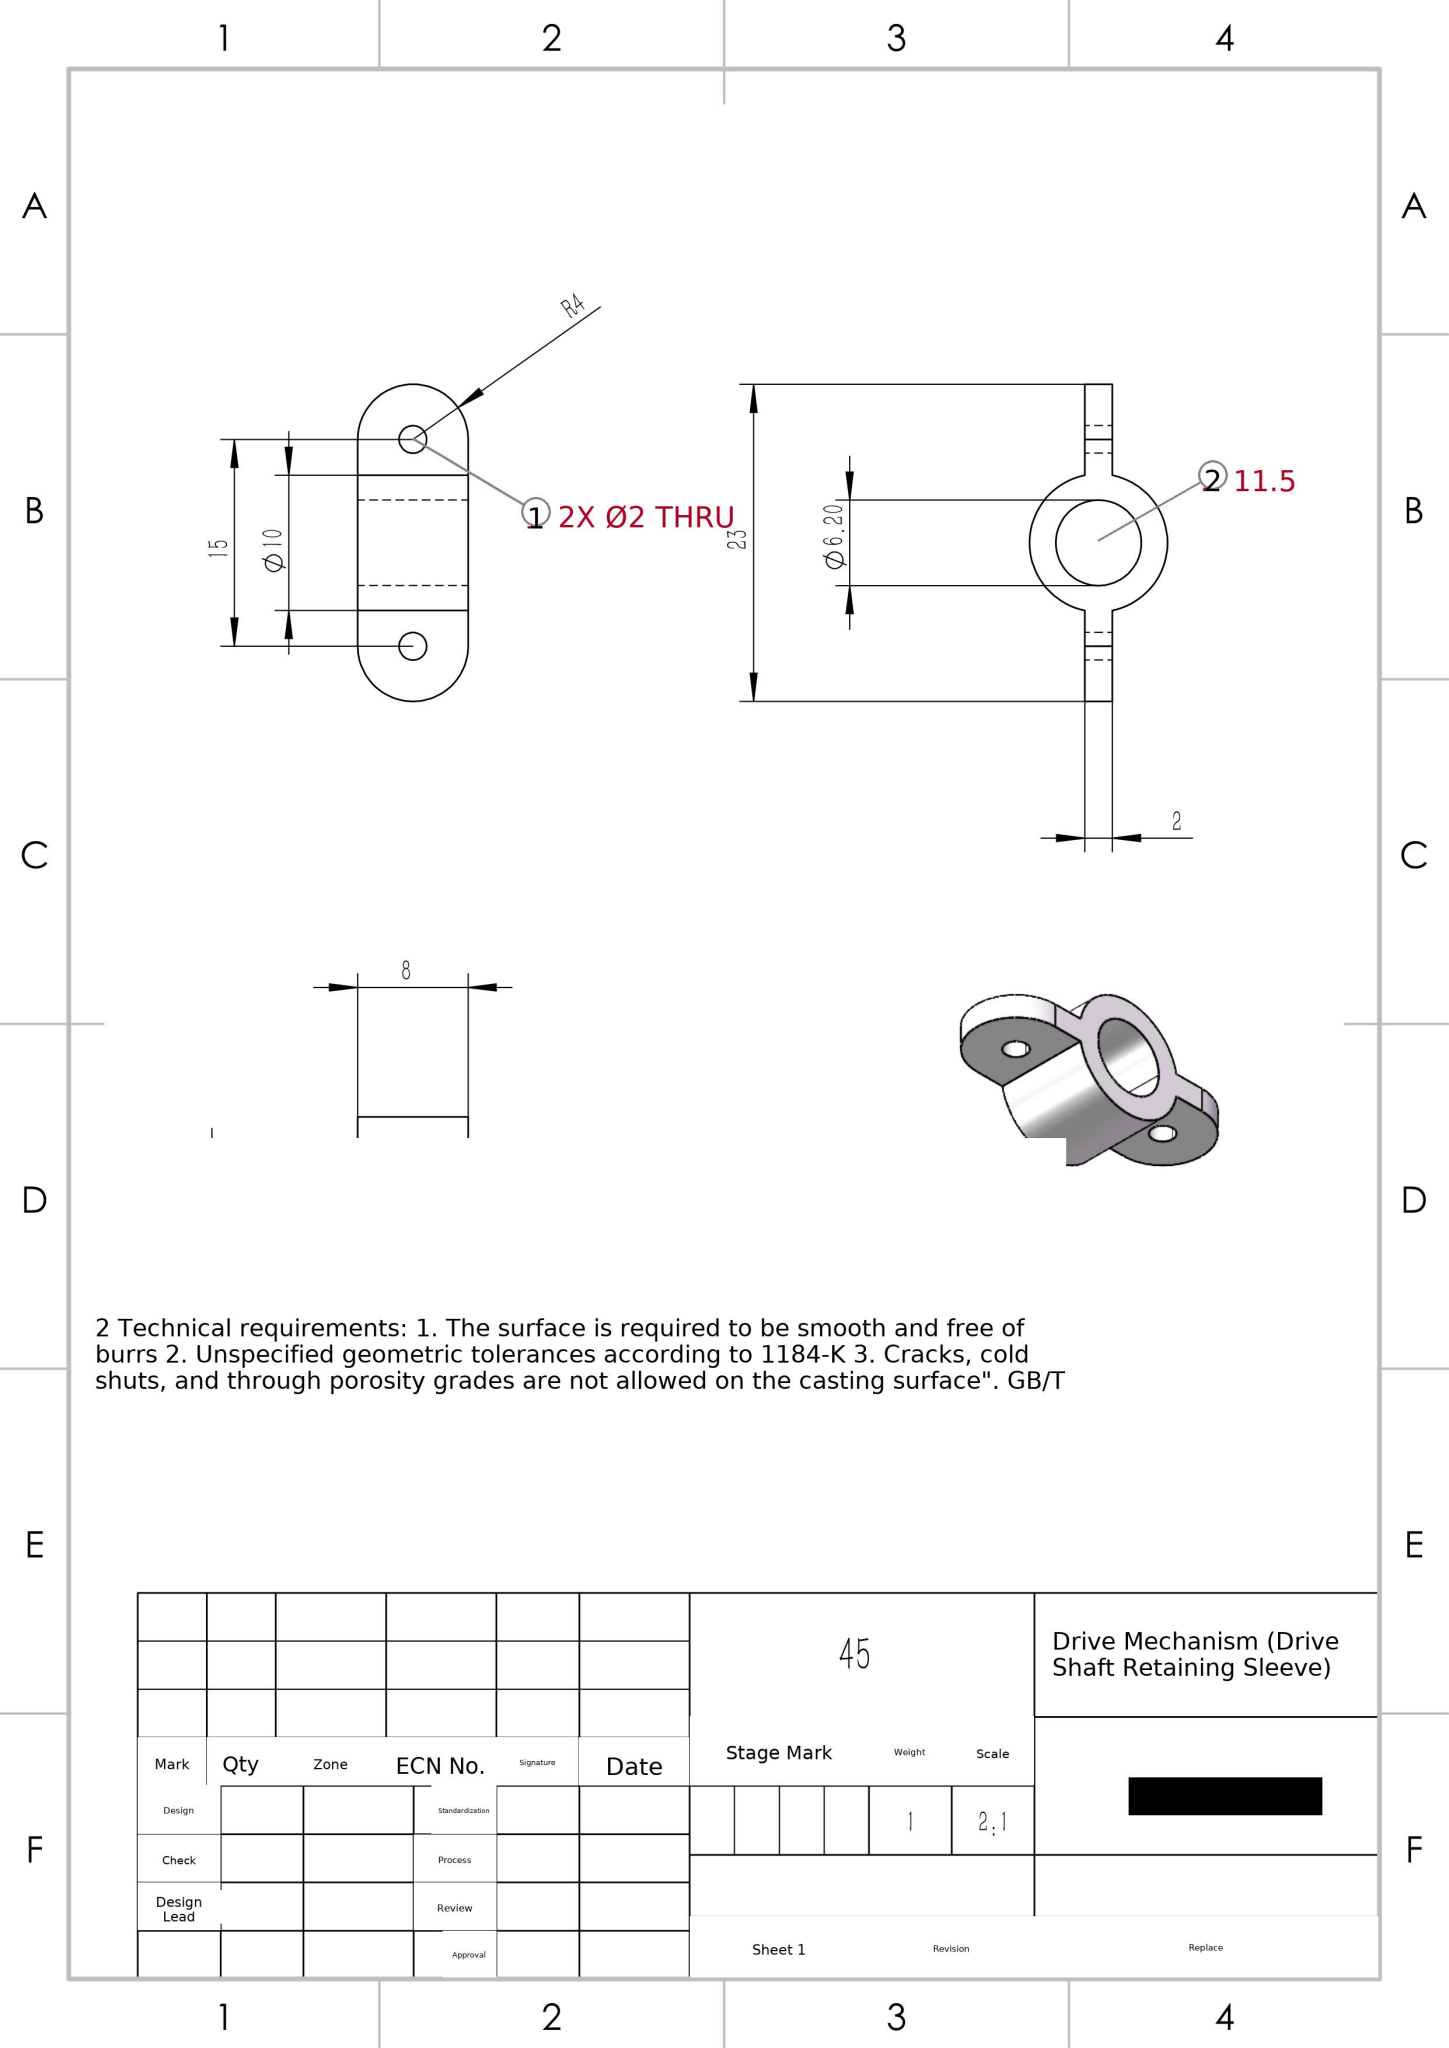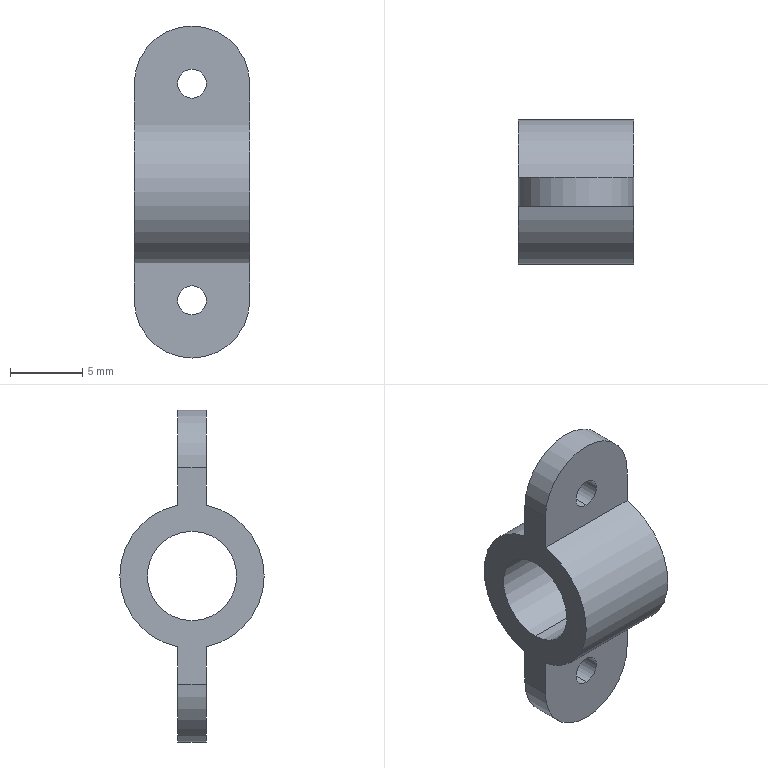Part | SolidWorks | mm | material 45 | 1 solid | 17 faces | box 8 x 10 x 23 mm | volume 556 mm3 | cylinder 11 | plane 6 | commonest cylinder face diameters 2 x4 8 x3 10 x2 6.2 x2
STEP:
#1=CARTESIAN_POINT('',(-4.,1.,-4.899));
#2=VERTEX_POINT('',#1);
#3=CARTESIAN_POINT('',(4.,1.,-4.899));
#4=VERTEX_POINT('',#3);
#5=CARTESIAN_POINT('',(4.,1.,-4.899));
#6=DIRECTION('',(1.,0.,0.));
#7=VECTOR('',#6,1000.);
#8=LINE('',#5,#7);
#9=EDGE_CURVE('',#2,#4,#8,.T.);
#10=ORIENTED_EDGE('',*,*,#9,.F.);
#11=CARTESIAN_POINT('',(-4.,1.,4.899));
#12=VERTEX_POINT('',#11);
#13=CARTESIAN_POINT('',(-4.,0.,0.));
#14=DIRECTION('',(1.,0.,0.));
#15=DIRECTION('',(0.,0.,-1.));
#16=AXIS2_PLACEMENT_3D('',#13,#14,#15);
#17=CIRCLE('',#16,5.);
#18=EDGE_CURVE('',#2,#12,#17,.T.);
#19=ORIENTED_EDGE('',*,*,#18,.T.);
#20=CARTESIAN_POINT('',(4.,1.,4.899));
#21=VERTEX_POINT('',#20);
#22=CARTESIAN_POINT('',(4.,1.,4.899));
#23=DIRECTION('',(-1.,0.,0.));
#24=VECTOR('',#23,1000.);
#25=LINE('',#22,#24);
#26=EDGE_CURVE('',#21,#12,#25,.T.);
#27=ORIENTED_EDGE('',*,*,#26,.F.);
#28=CARTESIAN_POINT('',(4.,0.,0.));
#29=DIRECTION('',(1.,0.,0.));
#30=DIRECTION('',(0.,0.,-1.));
#31=AXIS2_PLACEMENT_3D('',#28,#29,#30);
#32=CIRCLE('',#31,5.);
#33=EDGE_CURVE('',#4,#21,#32,.T.);
#34=ORIENTED_EDGE('',*,*,#33,.F.);
#35=EDGE_LOOP('',(#10,#19,#27,#34));
#36=FACE_OUTER_BOUND('',#35,.T.);
#37=CARTESIAN_POINT('',(4.,0.,0.));
#38=DIRECTION('',(-1.,0.,0.));
#39=DIRECTION('',(0.,0.,1.));
#40=AXIS2_PLACEMENT_3D('',#37,#38,#39);
#41=CYLINDRICAL_SURFACE('',#40,5.);
#42=ADVANCED_FACE('',(#36),#41,.T.);
#43=CARTESIAN_POINT('',(-4.,-1.,4.899));
#44=VERTEX_POINT('',#43);
#45=CARTESIAN_POINT('',(-4.,-1.,-4.899));
#46=VERTEX_POINT('',#45);
#47=CARTESIAN_POINT('',(-4.,0.,0.));
#48=DIRECTION('',(1.,0.,0.));
#49=DIRECTION('',(0.,0.,-1.));
#50=AXIS2_PLACEMENT_3D('',#47,#48,#49);
#51=CIRCLE('',#50,5.);
#52=EDGE_CURVE('',#44,#46,#51,.T.);
#53=ORIENTED_EDGE('',*,*,#52,.T.);
#54=CARTESIAN_POINT('',(4.,-1.,-4.899));
#55=VERTEX_POINT('',#54);
#56=CARTESIAN_POINT('',(4.,-1.,-4.899));
#57=DIRECTION('',(1.,0.,0.));
#58=VECTOR('',#57,1000.);
#59=LINE('',#56,#58);
#60=EDGE_CURVE('',#46,#55,#59,.T.);
#61=ORIENTED_EDGE('',*,*,#60,.T.);
#62=CARTESIAN_POINT('',(4.,-1.,4.899));
#63=VERTEX_POINT('',#62);
#64=CARTESIAN_POINT('',(4.,0.,0.));
#65=DIRECTION('',(1.,0.,0.));
#66=DIRECTION('',(0.,0.,-1.));
#67=AXIS2_PLACEMENT_3D('',#64,#65,#66);
#68=CIRCLE('',#67,5.);
#69=EDGE_CURVE('',#63,#55,#68,.T.);
#70=ORIENTED_EDGE('',*,*,#69,.F.);
#71=CARTESIAN_POINT('',(4.,-1.,4.899));
#72=DIRECTION('',(-1.,0.,0.));
#73=VECTOR('',#72,1000.);
#74=LINE('',#71,#73);
#75=EDGE_CURVE('',#63,#44,#74,.T.);
#76=ORIENTED_EDGE('',*,*,#75,.T.);
#77=EDGE_LOOP('',(#53,#61,#70,#76));
#78=FACE_OUTER_BOUND('',#77,.T.);
#79=CARTESIAN_POINT('',(4.,0.,0.));
#80=DIRECTION('',(-1.,0.,0.));
#81=DIRECTION('',(0.,0.,1.));
#82=AXIS2_PLACEMENT_3D('',#79,#80,#81);
#83=CYLINDRICAL_SURFACE('',#82,5.);
#84=ADVANCED_FACE('',(#78),#83,.T.);
#85=CARTESIAN_POINT('',(4.,0.,-3.1));
#86=VERTEX_POINT('',#85);
#87=CARTESIAN_POINT('',(-4.,0.,-3.1));
#88=VERTEX_POINT('',#87);
#89=CARTESIAN_POINT('',(4.,0.,-3.1));
#90=DIRECTION('',(-1.,0.,0.));
#91=VECTOR('',#90,1000.);
#92=LINE('',#89,#91);
#93=EDGE_CURVE('',#86,#88,#92,.T.);
#94=ORIENTED_EDGE('',*,*,#93,.F.);
#95=CARTESIAN_POINT('',(4.,0.,3.1));
#96=VERTEX_POINT('',#95);
#97=CARTESIAN_POINT('',(4.,0.,0.));
#98=DIRECTION('',(1.,0.,0.));
#99=DIRECTION('',(0.,0.,-1.));
#100=AXIS2_PLACEMENT_3D('',#97,#98,#99);
#101=CIRCLE('',#100,3.1);
#102=EDGE_CURVE('',#86,#96,#101,.T.);
#103=ORIENTED_EDGE('',*,*,#102,.T.);
#104=CARTESIAN_POINT('',(-4.,0.,3.1));
#105=VERTEX_POINT('',#104);
#106=CARTESIAN_POINT('',(4.,0.,3.1));
#107=DIRECTION('',(-1.,0.,0.));
#108=VECTOR('',#107,1000.);
#109=LINE('',#106,#108);
#110=EDGE_CURVE('',#96,#105,#109,.T.);
#111=ORIENTED_EDGE('',*,*,#110,.T.);
#112=CARTESIAN_POINT('',(-4.,0.,0.));
#113=DIRECTION('',(1.,0.,0.));
#114=DIRECTION('',(0.,0.,-1.));
#115=AXIS2_PLACEMENT_3D('',#112,#113,#114);
#116=CIRCLE('',#115,3.1);
#117=EDGE_CURVE('',#88,#105,#116,.T.);
#118=ORIENTED_EDGE('',*,*,#117,.F.);
#119=EDGE_LOOP('',(#94,#103,#111,#118));
#120=FACE_OUTER_BOUND('',#119,.T.);
#121=CARTESIAN_POINT('',(4.,0.,0.));
#122=DIRECTION('',(-1.,0.,0.));
#123=DIRECTION('',(0.,0.,1.));
#124=AXIS2_PLACEMENT_3D('',#121,#122,#123);
#125=CYLINDRICAL_SURFACE('',#124,3.1);
#126=ADVANCED_FACE('',(#120),#125,.F.);
#127=CARTESIAN_POINT('',(0.,1.,8.5));
#128=VERTEX_POINT('',#127);
#129=CARTESIAN_POINT('',(0.,-1.,8.5));
#130=VERTEX_POINT('',#129);
#131=CARTESIAN_POINT('',(0.,1.,8.5));
#132=DIRECTION('',(0.,-1.,0.));
#133=VECTOR('',#132,1000.);
#134=LINE('',#131,#133);
#135=EDGE_CURVE('',#128,#130,#134,.T.);
#136=ORIENTED_EDGE('',*,*,#135,.F.);
#137=CARTESIAN_POINT('',(0.,1.,6.5));
#138=VERTEX_POINT('',#137);
#139=CARTESIAN_POINT('',(0.,1.,7.5));
#140=DIRECTION('',(0.,1.,0.));
#141=DIRECTION('',(0.,0.,1.));
#142=AXIS2_PLACEMENT_3D('',#139,#140,#141);
#143=CIRCLE('',#142,1.);
#144=EDGE_CURVE('',#128,#138,#143,.T.);
#145=ORIENTED_EDGE('',*,*,#144,.T.);
#146=CARTESIAN_POINT('',(0.,-1.,6.5));
#147=VERTEX_POINT('',#146);
#148=CARTESIAN_POINT('',(0.,1.,6.5));
#149=DIRECTION('',(0.,-1.,0.));
#150=VECTOR('',#149,1000.);
#151=LINE('',#148,#150);
#152=EDGE_CURVE('',#138,#147,#151,.T.);
#153=ORIENTED_EDGE('',*,*,#152,.T.);
#154=CARTESIAN_POINT('',(0.,-1.,7.5));
#155=DIRECTION('',(0.,1.,0.));
#156=DIRECTION('',(0.,0.,1.));
#157=AXIS2_PLACEMENT_3D('',#154,#155,#156);
#158=CIRCLE('',#157,1.);
#159=EDGE_CURVE('',#130,#147,#158,.T.);
#160=ORIENTED_EDGE('',*,*,#159,.F.);
#161=EDGE_LOOP('',(#136,#145,#153,#160));
#162=FACE_OUTER_BOUND('',#161,.T.);
#163=CARTESIAN_POINT('',(0.,1.,7.5));
#164=DIRECTION('',(0.,-1.,0.));
#165=DIRECTION('',(0.,0.,-1.));
#166=AXIS2_PLACEMENT_3D('',#163,#164,#165);
#167=CYLINDRICAL_SURFACE('',#166,1.);
#168=ADVANCED_FACE('',(#162),#167,.F.);
#169=CARTESIAN_POINT('',(0.,1.,-6.5));
#170=VERTEX_POINT('',#169);
#171=CARTESIAN_POINT('',(0.,-1.,-6.5));
#172=VERTEX_POINT('',#171);
#173=CARTESIAN_POINT('',(0.,1.,-6.5));
#174=DIRECTION('',(0.,-1.,0.));
#175=VECTOR('',#174,1000.);
#176=LINE('',#173,#175);
#177=EDGE_CURVE('',#170,#172,#176,.T.);
#178=ORIENTED_EDGE('',*,*,#177,.F.);
#179=CARTESIAN_POINT('',(0.,1.,-8.5));
#180=VERTEX_POINT('',#179);
#181=CARTESIAN_POINT('',(0.,1.,-7.5));
#182=DIRECTION('',(0.,1.,0.));
#183=DIRECTION('',(0.,0.,1.));
#184=AXIS2_PLACEMENT_3D('',#181,#182,#183);
#185=CIRCLE('',#184,1.);
#186=EDGE_CURVE('',#170,#180,#185,.T.);
#187=ORIENTED_EDGE('',*,*,#186,.T.);
#188=CARTESIAN_POINT('',(0.,-1.,-8.5));
#189=VERTEX_POINT('',#188);
#190=CARTESIAN_POINT('',(0.,1.,-8.5));
#191=DIRECTION('',(0.,-1.,0.));
#192=VECTOR('',#191,1000.);
#193=LINE('',#190,#192);
#194=EDGE_CURVE('',#180,#189,#193,.T.);
#195=ORIENTED_EDGE('',*,*,#194,.T.);
#196=CARTESIAN_POINT('',(0.,-1.,-7.5));
#197=DIRECTION('',(0.,1.,0.));
#198=DIRECTION('',(0.,0.,1.));
#199=AXIS2_PLACEMENT_3D('',#196,#197,#198);
#200=CIRCLE('',#199,1.);
#201=EDGE_CURVE('',#172,#189,#200,.T.);
#202=ORIENTED_EDGE('',*,*,#201,.F.);
#203=EDGE_LOOP('',(#178,#187,#195,#202));
#204=FACE_OUTER_BOUND('',#203,.T.);
#205=CARTESIAN_POINT('',(0.,1.,-7.5));
#206=DIRECTION('',(0.,-1.,0.));
#207=DIRECTION('',(0.,0.,-1.));
#208=AXIS2_PLACEMENT_3D('',#205,#206,#207);
#209=CYLINDRICAL_SURFACE('',#208,1.);
#210=ADVANCED_FACE('',(#204),#209,.F.);
#211=CARTESIAN_POINT('',(-4.,0.,0.));
#212=DIRECTION('',(1.,0.,0.));
#213=DIRECTION('',(0.,0.,-1.));
#214=AXIS2_PLACEMENT_3D('',#211,#212,#213);
#215=CIRCLE('',#214,3.1);
#216=EDGE_CURVE('',#105,#88,#215,.T.);
#217=ORIENTED_EDGE('',*,*,#216,.T.);
#218=ORIENTED_EDGE('',*,*,#117,.T.);
#219=EDGE_LOOP('',(#217,#218));
#220=FACE_BOUND('',#219,.T.);
#221=CARTESIAN_POINT('',(-4.,1.,7.5));
#222=VERTEX_POINT('',#221);
#223=CARTESIAN_POINT('',(-4.,1.,7.5));
#224=DIRECTION('',(0.,0.,1.));
#225=VECTOR('',#224,1000.);
#226=LINE('',#223,#225);
#227=EDGE_CURVE('',#12,#222,#226,.T.);
#228=ORIENTED_EDGE('',*,*,#227,.F.);
#229=ORIENTED_EDGE('',*,*,#18,.F.);
#230=CARTESIAN_POINT('',(-4.,1.,-7.5));
#231=VERTEX_POINT('',#230);
#232=CARTESIAN_POINT('',(-4.,1.,7.5));
#233=DIRECTION('',(0.,0.,1.));
#234=VECTOR('',#233,1000.);
#235=LINE('',#232,#234);
#236=EDGE_CURVE('',#231,#2,#235,.T.);
#237=ORIENTED_EDGE('',*,*,#236,.F.);
#238=CARTESIAN_POINT('',(-4.,-1.,-7.5));
#239=VERTEX_POINT('',#238);
#240=CARTESIAN_POINT('',(-4.,1.,-7.5));
#241=DIRECTION('',(0.,-1.,0.));
#242=VECTOR('',#241,1000.);
#243=LINE('',#240,#242);
#244=EDGE_CURVE('',#231,#239,#243,.T.);
#245=ORIENTED_EDGE('',*,*,#244,.T.);
#246=CARTESIAN_POINT('',(-4.,-1.,7.5));
#247=DIRECTION('',(0.,0.,1.));
#248=VECTOR('',#247,1000.);
#249=LINE('',#246,#248);
#250=EDGE_CURVE('',#239,#46,#249,.T.);
#251=ORIENTED_EDGE('',*,*,#250,.T.);
#252=ORIENTED_EDGE('',*,*,#52,.F.);
#253=CARTESIAN_POINT('',(-4.,-1.,7.5));
#254=VERTEX_POINT('',#253);
#255=CARTESIAN_POINT('',(-4.,-1.,7.5));
#256=DIRECTION('',(0.,0.,1.));
#257=VECTOR('',#256,1000.);
#258=LINE('',#255,#257);
#259=EDGE_CURVE('',#44,#254,#258,.T.);
#260=ORIENTED_EDGE('',*,*,#259,.T.);
#261=CARTESIAN_POINT('',(-4.,1.,7.5));
#262=DIRECTION('',(0.,-1.,0.));
#263=VECTOR('',#262,1000.);
#264=LINE('',#261,#263);
#265=EDGE_CURVE('',#222,#254,#264,.T.);
#266=ORIENTED_EDGE('',*,*,#265,.F.);
#267=EDGE_LOOP('',(#228,#229,#237,#245,#251,#252,#260,#266));
#268=FACE_OUTER_BOUND('',#267,.T.);
#269=CARTESIAN_POINT('',(-4.,1.,7.5));
#270=DIRECTION('',(1.,0.,0.));
#271=DIRECTION('',(0.,1.,0.));
#272=AXIS2_PLACEMENT_3D('',#269,#270,#271);
#273=PLANE('',#272);
#274=ADVANCED_FACE('',(#220,#268),#273,.F.);
#275=CARTESIAN_POINT('',(0.,1.,-11.5));
#276=VERTEX_POINT('',#275);
#277=CARTESIAN_POINT('',(0.,-1.,-11.5));
#278=VERTEX_POINT('',#277);
#279=CARTESIAN_POINT('',(0.,1.,-11.5));
#280=DIRECTION('',(0.,-1.,0.));
#281=VECTOR('',#280,1000.);
#282=LINE('',#279,#281);
#283=EDGE_CURVE('',#276,#278,#282,.T.);
#284=ORIENTED_EDGE('',*,*,#283,.F.);
#285=CARTESIAN_POINT('',(4.,1.,-7.5));
#286=VERTEX_POINT('',#285);
#287=CARTESIAN_POINT('',(0.,1.,-7.5));
#288=DIRECTION('',(0.,1.,0.));
#289=DIRECTION('',(0.,0.,1.));
#290=AXIS2_PLACEMENT_3D('',#287,#288,#289);
#291=CIRCLE('',#290,4.);
#292=EDGE_CURVE('',#286,#276,#291,.T.);
#293=ORIENTED_EDGE('',*,*,#292,.F.);
#294=CARTESIAN_POINT('',(4.,-1.,-7.5));
#295=VERTEX_POINT('',#294);
#296=CARTESIAN_POINT('',(4.,1.,-7.5));
#297=DIRECTION('',(0.,-1.,0.));
#298=VECTOR('',#297,1000.);
#299=LINE('',#296,#298);
#300=EDGE_CURVE('',#286,#295,#299,.T.);
#301=ORIENTED_EDGE('',*,*,#300,.T.);
#302=CARTESIAN_POINT('',(0.,-1.,-7.5));
#303=DIRECTION('',(0.,1.,0.));
#304=DIRECTION('',(0.,0.,1.));
#305=AXIS2_PLACEMENT_3D('',#302,#303,#304);
#306=CIRCLE('',#305,4.);
#307=EDGE_CURVE('',#295,#278,#306,.T.);
#308=ORIENTED_EDGE('',*,*,#307,.T.);
#309=EDGE_LOOP('',(#284,#293,#301,#308));
#310=FACE_OUTER_BOUND('',#309,.T.);
#311=CARTESIAN_POINT('',(0.,1.,-7.5));
#312=DIRECTION('',(0.,-1.,0.));
#313=DIRECTION('',(0.,0.,-1.));
#314=AXIS2_PLACEMENT_3D('',#311,#312,#313);
#315=CYLINDRICAL_SURFACE('',#314,4.);
#316=ADVANCED_FACE('',(#310),#315,.T.);
#317=CARTESIAN_POINT('',(4.,0.,0.));
#318=DIRECTION('',(1.,0.,0.));
#319=DIRECTION('',(0.,0.,-1.));
#320=AXIS2_PLACEMENT_3D('',#317,#318,#319);
#321=CIRCLE('',#320,3.1);
#322=EDGE_CURVE('',#96,#86,#321,.T.);
#323=ORIENTED_EDGE('',*,*,#322,.F.);
#324=ORIENTED_EDGE('',*,*,#102,.F.);
#325=EDGE_LOOP('',(#323,#324));
#326=FACE_BOUND('',#325,.T.);
#327=CARTESIAN_POINT('',(4.,-1.,7.5));
#328=VERTEX_POINT('',#327);
#329=CARTESIAN_POINT('',(4.,-1.,7.5));
#330=DIRECTION('',(0.,0.,-1.));
#331=VECTOR('',#330,1000.);
#332=LINE('',#329,#331);
#333=EDGE_CURVE('',#328,#63,#332,.T.);
#334=ORIENTED_EDGE('',*,*,#333,.T.);
#335=ORIENTED_EDGE('',*,*,#69,.T.);
#336=CARTESIAN_POINT('',(4.,-1.,7.5));
#337=DIRECTION('',(0.,0.,-1.));
#338=VECTOR('',#337,1000.);
#339=LINE('',#336,#338);
#340=EDGE_CURVE('',#55,#295,#339,.T.);
#341=ORIENTED_EDGE('',*,*,#340,.T.);
#342=ORIENTED_EDGE('',*,*,#300,.F.);
#343=CARTESIAN_POINT('',(4.,1.,7.5));
#344=DIRECTION('',(0.,0.,-1.));
#345=VECTOR('',#344,1000.);
#346=LINE('',#343,#345);
#347=EDGE_CURVE('',#4,#286,#346,.T.);
#348=ORIENTED_EDGE('',*,*,#347,.F.);
#349=ORIENTED_EDGE('',*,*,#33,.T.);
#350=CARTESIAN_POINT('',(4.,1.,7.5));
#351=VERTEX_POINT('',#350);
#352=CARTESIAN_POINT('',(4.,1.,7.5));
#353=DIRECTION('',(0.,0.,-1.));
#354=VECTOR('',#353,1000.);
#355=LINE('',#352,#354);
#356=EDGE_CURVE('',#351,#21,#355,.T.);
#357=ORIENTED_EDGE('',*,*,#356,.F.);
#358=CARTESIAN_POINT('',(4.,1.,7.5));
#359=DIRECTION('',(0.,-1.,0.));
#360=VECTOR('',#359,1000.);
#361=LINE('',#358,#360);
#362=EDGE_CURVE('',#351,#328,#361,.T.);
#363=ORIENTED_EDGE('',*,*,#362,.T.);
#364=EDGE_LOOP('',(#334,#335,#341,#342,#348,#349,#357,#363));
#365=FACE_OUTER_BOUND('',#364,.T.);
#366=CARTESIAN_POINT('',(4.,1.,7.5));
#367=DIRECTION('',(-1.,0.,0.));
#368=DIRECTION('',(0.,0.,1.));
#369=AXIS2_PLACEMENT_3D('',#366,#367,#368);
#370=PLANE('',#369);
#371=ADVANCED_FACE('',(#326,#365),#370,.F.);
#372=CARTESIAN_POINT('',(0.,-1.,7.5));
#373=DIRECTION('',(0.,1.,0.));
#374=DIRECTION('',(0.,0.,1.));
#375=AXIS2_PLACEMENT_3D('',#372,#373,#374);
#376=CIRCLE('',#375,4.);
#377=EDGE_CURVE('',#254,#328,#376,.T.);
#378=ORIENTED_EDGE('',*,*,#377,.T.);
#379=ORIENTED_EDGE('',*,*,#362,.F.);
#380=CARTESIAN_POINT('',(0.,1.,7.5));
#381=DIRECTION('',(0.,1.,0.));
#382=DIRECTION('',(0.,0.,1.));
#383=AXIS2_PLACEMENT_3D('',#380,#381,#382);
#384=CIRCLE('',#383,4.);
#385=EDGE_CURVE('',#222,#351,#384,.T.);
#386=ORIENTED_EDGE('',*,*,#385,.F.);
#387=ORIENTED_EDGE('',*,*,#265,.T.);
#388=EDGE_LOOP('',(#378,#379,#386,#387));
#389=FACE_OUTER_BOUND('',#388,.T.);
#390=CARTESIAN_POINT('',(0.,1.,7.5));
#391=DIRECTION('',(0.,-1.,0.));
#392=DIRECTION('',(0.,0.,-1.));
#393=AXIS2_PLACEMENT_3D('',#390,#391,#392);
#394=CYLINDRICAL_SURFACE('',#393,4.);
#395=ADVANCED_FACE('',(#389),#394,.T.);
#396=CARTESIAN_POINT('',(0.,-1.,7.5));
#397=DIRECTION('',(0.,1.,0.));
#398=DIRECTION('',(0.,0.,1.));
#399=AXIS2_PLACEMENT_3D('',#396,#397,#398);
#400=CIRCLE('',#399,1.);
#401=EDGE_CURVE('',#147,#130,#400,.T.);
#402=ORIENTED_EDGE('',*,*,#401,.T.);
#403=ORIENTED_EDGE('',*,*,#159,.T.);
#404=EDGE_LOOP('',(#402,#403));
#405=FACE_BOUND('',#404,.T.);
#406=ORIENTED_EDGE('',*,*,#75,.F.);
#407=ORIENTED_EDGE('',*,*,#333,.F.);
#408=ORIENTED_EDGE('',*,*,#377,.F.);
#409=ORIENTED_EDGE('',*,*,#259,.F.);
#410=EDGE_LOOP('',(#406,#407,#408,#409));
#411=FACE_OUTER_BOUND('',#410,.T.);
#412=CARTESIAN_POINT('',(0.,-1.,7.5));
#413=DIRECTION('',(0.,1.,0.));
#414=DIRECTION('',(1.,0.,0.));
#415=AXIS2_PLACEMENT_3D('',#412,#413,#414);
#416=PLANE('',#415);
#417=ADVANCED_FACE('',(#405,#411),#416,.F.);
#418=CARTESIAN_POINT('',(0.,-1.,-7.5));
#419=DIRECTION('',(0.,1.,0.));
#420=DIRECTION('',(0.,0.,1.));
#421=AXIS2_PLACEMENT_3D('',#418,#419,#420);
#422=CIRCLE('',#421,1.);
#423=EDGE_CURVE('',#189,#172,#422,.T.);
#424=ORIENTED_EDGE('',*,*,#423,.T.);
#425=ORIENTED_EDGE('',*,*,#201,.T.);
#426=EDGE_LOOP('',(#424,#425));
#427=FACE_BOUND('',#426,.T.);
#428=ORIENTED_EDGE('',*,*,#60,.F.);
#429=ORIENTED_EDGE('',*,*,#250,.F.);
#430=CARTESIAN_POINT('',(0.,-1.,-7.5));
#431=DIRECTION('',(0.,1.,0.));
#432=DIRECTION('',(0.,0.,1.));
#433=AXIS2_PLACEMENT_3D('',#430,#431,#432);
#434=CIRCLE('',#433,4.);
#435=EDGE_CURVE('',#278,#239,#434,.T.);
#436=ORIENTED_EDGE('',*,*,#435,.F.);
#437=ORIENTED_EDGE('',*,*,#307,.F.);
#438=ORIENTED_EDGE('',*,*,#340,.F.);
#439=EDGE_LOOP('',(#428,#429,#436,#437,#438));
#440=FACE_OUTER_BOUND('',#439,.T.);
#441=CARTESIAN_POINT('',(0.,-1.,7.5));
#442=DIRECTION('',(0.,1.,0.));
#443=DIRECTION('',(1.,0.,0.));
#444=AXIS2_PLACEMENT_3D('',#441,#442,#443);
#445=PLANE('',#444);
#446=ADVANCED_FACE('',(#427,#440),#445,.F.);
#447=CARTESIAN_POINT('',(0.,1.,7.5));
#448=DIRECTION('',(0.,1.,0.));
#449=DIRECTION('',(0.,0.,1.));
#450=AXIS2_PLACEMENT_3D('',#447,#448,#449);
#451=CIRCLE('',#450,1.);
#452=EDGE_CURVE('',#138,#128,#451,.T.);
#453=ORIENTED_EDGE('',*,*,#452,.F.);
#454=ORIENTED_EDGE('',*,*,#144,.F.);
#455=EDGE_LOOP('',(#453,#454));
#456=FACE_BOUND('',#455,.T.);
#457=ORIENTED_EDGE('',*,*,#356,.T.);
#458=ORIENTED_EDGE('',*,*,#26,.T.);
#459=ORIENTED_EDGE('',*,*,#227,.T.);
#460=ORIENTED_EDGE('',*,*,#385,.T.);
#461=EDGE_LOOP('',(#457,#458,#459,#460));
#462=FACE_OUTER_BOUND('',#461,.T.);
#463=CARTESIAN_POINT('',(0.,1.,7.5));
#464=DIRECTION('',(0.,1.,0.));
#465=DIRECTION('',(1.,0.,0.));
#466=AXIS2_PLACEMENT_3D('',#463,#464,#465);
#467=PLANE('',#466);
#468=ADVANCED_FACE('',(#456,#462),#467,.T.);
#469=CARTESIAN_POINT('',(0.,1.,-7.5));
#470=DIRECTION('',(0.,1.,0.));
#471=DIRECTION('',(0.,0.,1.));
#472=AXIS2_PLACEMENT_3D('',#469,#470,#471);
#473=CIRCLE('',#472,1.);
#474=EDGE_CURVE('',#180,#170,#473,.T.);
#475=ORIENTED_EDGE('',*,*,#474,.F.);
#476=ORIENTED_EDGE('',*,*,#186,.F.);
#477=EDGE_LOOP('',(#475,#476));
#478=FACE_BOUND('',#477,.T.);
#479=ORIENTED_EDGE('',*,*,#236,.T.);
#480=ORIENTED_EDGE('',*,*,#9,.T.);
#481=ORIENTED_EDGE('',*,*,#347,.T.);
#482=ORIENTED_EDGE('',*,*,#292,.T.);
#483=CARTESIAN_POINT('',(0.,1.,-7.5));
#484=DIRECTION('',(0.,1.,0.));
#485=DIRECTION('',(0.,0.,1.));
#486=AXIS2_PLACEMENT_3D('',#483,#484,#485);
#487=CIRCLE('',#486,4.);
#488=EDGE_CURVE('',#276,#231,#487,.T.);
#489=ORIENTED_EDGE('',*,*,#488,.T.);
#490=EDGE_LOOP('',(#479,#480,#481,#482,#489));
#491=FACE_OUTER_BOUND('',#490,.T.);
#492=CARTESIAN_POINT('',(0.,1.,7.5));
#493=DIRECTION('',(0.,1.,0.));
#494=DIRECTION('',(1.,0.,0.));
#495=AXIS2_PLACEMENT_3D('',#492,#493,#494);
#496=PLANE('',#495);
#497=ADVANCED_FACE('',(#478,#491),#496,.T.);
#498=ORIENTED_EDGE('',*,*,#488,.F.);
#499=ORIENTED_EDGE('',*,*,#283,.T.);
#500=ORIENTED_EDGE('',*,*,#435,.T.);
#501=ORIENTED_EDGE('',*,*,#244,.F.);
#502=EDGE_LOOP('',(#498,#499,#500,#501));
#503=FACE_OUTER_BOUND('',#502,.T.);
#504=CARTESIAN_POINT('',(0.,1.,-7.5));
#505=DIRECTION('',(0.,-1.,0.));
#506=DIRECTION('',(0.,0.,-1.));
#507=AXIS2_PLACEMENT_3D('',#504,#505,#506);
#508=CYLINDRICAL_SURFACE('',#507,4.);
#509=ADVANCED_FACE('',(#503),#508,.T.);
#510=ORIENTED_EDGE('',*,*,#474,.T.);
#511=ORIENTED_EDGE('',*,*,#177,.T.);
#512=ORIENTED_EDGE('',*,*,#423,.F.);
#513=ORIENTED_EDGE('',*,*,#194,.F.);
#514=EDGE_LOOP('',(#510,#511,#512,#513));
#515=FACE_OUTER_BOUND('',#514,.T.);
#516=CARTESIAN_POINT('',(0.,1.,-7.5));
#517=DIRECTION('',(0.,-1.,0.));
#518=DIRECTION('',(0.,0.,-1.));
#519=AXIS2_PLACEMENT_3D('',#516,#517,#518);
#520=CYLINDRICAL_SURFACE('',#519,1.);
#521=ADVANCED_FACE('',(#515),#520,.F.);
#522=ORIENTED_EDGE('',*,*,#452,.T.);
#523=ORIENTED_EDGE('',*,*,#135,.T.);
#524=ORIENTED_EDGE('',*,*,#401,.F.);
#525=ORIENTED_EDGE('',*,*,#152,.F.);
#526=EDGE_LOOP('',(#522,#523,#524,#525));
#527=FACE_OUTER_BOUND('',#526,.T.);
#528=CARTESIAN_POINT('',(0.,1.,7.5));
#529=DIRECTION('',(0.,-1.,0.));
#530=DIRECTION('',(0.,0.,-1.));
#531=AXIS2_PLACEMENT_3D('',#528,#529,#530);
#532=CYLINDRICAL_SURFACE('',#531,1.);
#533=ADVANCED_FACE('',(#527),#532,.F.);
#534=ORIENTED_EDGE('',*,*,#322,.T.);
#535=ORIENTED_EDGE('',*,*,#93,.T.);
#536=ORIENTED_EDGE('',*,*,#216,.F.);
#537=ORIENTED_EDGE('',*,*,#110,.F.);
#538=EDGE_LOOP('',(#534,#535,#536,#537));
#539=FACE_OUTER_BOUND('',#538,.T.);
#540=CARTESIAN_POINT('',(4.,0.,0.));
#541=DIRECTION('',(-1.,0.,0.));
#542=DIRECTION('',(0.,0.,1.));
#543=AXIS2_PLACEMENT_3D('',#540,#541,#542);
#544=CYLINDRICAL_SURFACE('',#543,3.1);
#545=ADVANCED_FACE('',(#539),#544,.F.);
#546=CLOSED_SHELL('',(#42,#84,#126,#168,#210,#274,#316,#371,#395,#417,#446,#468,#497,#509,#521,#533,#545));
#547=MANIFOLD_SOLID_BREP('',#546);
#548=CARTESIAN_POINT('',(0.,0.,0.));
#549=DIRECTION('',(0.,0.,1.));
#550=DIRECTION('',(1.,0.,0.));
#551=AXIS2_PLACEMENT_3D('',#548,#549,#550);
#552=(LENGTH_UNIT()NAMED_UNIT(*)SI_UNIT(.MILLI.,.METRE.));
#553=UNCERTAINTY_MEASURE_WITH_UNIT(LENGTH_MEASURE(0.00001),#552,'','');
#554=(NAMED_UNIT(*)PLANE_ANGLE_UNIT()SI_UNIT($,.RADIAN.));
#555=(NAMED_UNIT(*)SI_UNIT($,.STERADIAN.)SOLID_ANGLE_UNIT());
#556=(GEOMETRIC_REPRESENTATION_CONTEXT(3)GLOBAL_UNCERTAINTY_ASSIGNED_CONTEXT((#553))GLOBAL_UNIT_ASSIGNED_CONTEXT((#552,#554,#555))REPRESENTATION_CONTEXT('',''));
#557=ADVANCED_BREP_SHAPE_REPRESENTATION('',(#547,#551),#556);